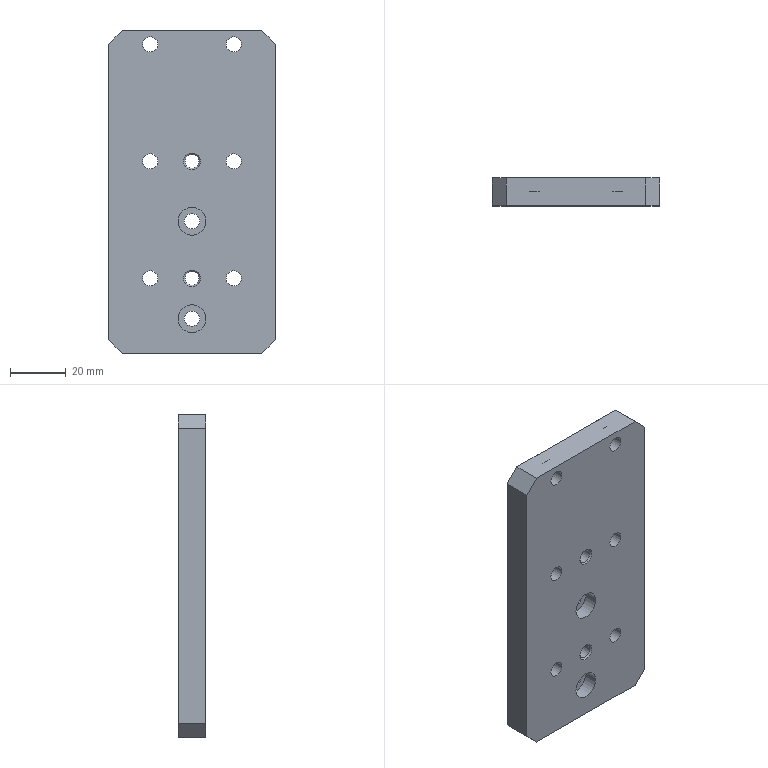Component | SolidWorks | 03-MillingMaterialMotorMountingPlate-1 | 1 solid | 62 faces | box 60 x 10 x 116 mm | volume 64612 mm3 | cylinder 36 | plane 18 | cone 8 | commonest cylinder face diameters 5.5 x16 9.99 x12 10 x4 5 x4
build123d program:
from build123d import *

# Parameters (mm, degrees)
SKETCH1_W                                            = 60
SKETCH1_H                                            = 116
EXTRUDE1_DEPTH                                       = 10
COUNTERBORE_FOR_M5_HEX_SOCKET_HEAD_CAP_S_D           = 5.5
COUNTERBORE_FOR_M5_HEX_SOCKET_HEAD_CAP_S_CBORE_D     = 9.99
COUNTERBORE_FOR_M5_HEX_SOCKET_HEAD_CAP_S_CBORE_DEPTH = 5
SKETCH4_R                                            = 2.5
EXTRUDE2_DEPTH                                       = 67.061
CHAMFER1_SIZE                                        = 0.5
CHAMFER2_SIZE                                        = 5
COUNTERBORE_FOR_M5_HEX_SOCKET_HEAD_C_2_D             = 5.5
COUNTERBORE_FOR_M5_HEX_SOCKET_HEAD_C_2_CBORE_D       = 10
COUNTERBORE_FOR_M5_HEX_SOCKET_HEAD_C_2_CBORE_DEPTH   = 5


with BuildPart() as part:
    # Sketch1 → Extrude1 (new body)
    with BuildSketch(Plane.XY):
        Rectangle(SKETCH1_W, SKETCH1_H)
    extrude(amount=EXTRUDE1_DEPTH)

    # Counterbore for M5 Hex Socket Head Cap S (through all)
    with Locations(Plane.XY.offset(10)):
        with Locations((15, 31), (-15, 31), (-15, -53), (15, -53), (-15, -11), (15, -11)):
            CounterBoreHole(COUNTERBORE_FOR_M5_HEX_SOCKET_HEAD_CAP_S_D / 2, COUNTERBORE_FOR_M5_HEX_SOCKET_HEAD_CAP_S_CBORE_D / 2, COUNTERBORE_FOR_M5_HEX_SOCKET_HEAD_CAP_S_CBORE_DEPTH)

    # Sketch4 → Extrude2 (cut, through all)
    with BuildSketch(Plane.XY.offset(10)):
        with Locations((0, 31)):
            Circle(SKETCH4_R)
        with Locations((0, -11)):
            Circle(SKETCH4_R)
    extrude(amount=-EXTRUDE2_DEPTH, mode=Mode.SUBTRACT)

    # Chamfer1
    chamfer1_edges = [part.edges().sort_by_distance(p)[0] for p in [
        (-2.5, 31, 0),
        (-2.5, 31, 10),
        (-2.5, -11, 0),
        (-2.5, -11, 10),
    ]]
    chamfer(chamfer1_edges, length=CHAMFER1_SIZE)

    # Chamfer2
    chamfer2_edges = [part.edges().sort_by_distance(p)[0] for p in [
        (30, -58, 5),
        (-30, -58, 5),
        (-30, 58, 5),
        (30, 58, 5),
    ]]
    chamfer(chamfer2_edges, length=CHAMFER2_SIZE)

    # Counterbore for M5 Hex Socket Head C 2 (through all)
    with Locations(Plane(origin=(0, 0, 0), x_dir=(-1, 0, 0), z_dir=(0, 0, -1))):
        with Locations((0, 10.5), (0, 45.5)):
            CounterBoreHole(COUNTERBORE_FOR_M5_HEX_SOCKET_HEAD_C_2_D / 2, COUNTERBORE_FOR_M5_HEX_SOCKET_HEAD_C_2_CBORE_D / 2, COUNTERBORE_FOR_M5_HEX_SOCKET_HEAD_C_2_CBORE_DEPTH)


solid = part.part

# Placed as in the assembly
solid = solid.moved(Location((0, 46, -104.197), (-90, 0, 0)))